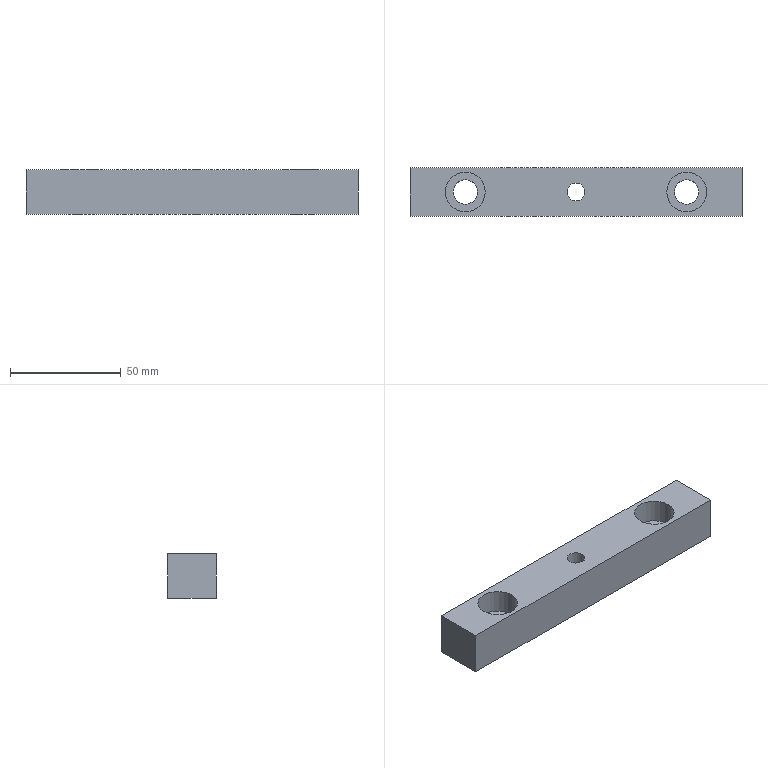Component | NX | DATUM_BLOCK | 1 solid | 13 faces | box 150 x 22 x 20 mm | volume 57750 mm3 | plane 8 | cylinder 5 | commonest cylinder face diameters 11 x2 18 x2 8 x1
STEP:
#1=CARTESIAN_POINT('',(0.,0.,0.));
#2=DIRECTION('',(0.,0.,1.));
#3=DIRECTION('',(1.,0.,0.));
#4=AXIS2_PLACEMENT_3D('',#1,#2,#3);
#5=CARTESIAN_POINT('',(-75.,-25.5,55.));
#6=VERTEX_POINT('',#5);
#7=CARTESIAN_POINT('',(-75.,-47.5,55.));
#8=VERTEX_POINT('',#7);
#9=CARTESIAN_POINT('',(-75.,-25.5,55.));
#10=DIRECTION('',(0.,-1.,0.));
#11=VECTOR('',#10,1.);
#12=LINE('',#9,#11);
#13=CARTESIAN_POINT('',(-75.,-25.5,35.));
#14=DIRECTION('',(-1.,0.,0.));
#15=DIRECTION('',(0.,0.,1.));
#16=AXIS2_PLACEMENT_3D('',#13,#14,#15);
#17=PLANE('',#16);
#18=CARTESIAN_POINT('',(20.,0.));
#19=DIRECTION('',(0.,-1.));
#20=VECTOR('',#19,1.);
#21=LINE('',#18,#20);
#22=(GEOMETRIC_REPRESENTATION_CONTEXT(2)PARAMETRIC_REPRESENTATION_CONTEXT()REPRESENTATION_CONTEXT('',''));
#23=DEFINITIONAL_REPRESENTATION('',(#21),#22);
#24=PCURVE('',#17,#23);
#25=CARTESIAN_POINT('',(0.,-36.5,55.));
#26=DIRECTION('',(0.,0.,1.));
#27=DIRECTION('',(1.,0.,0.));
#28=AXIS2_PLACEMENT_3D('',#25,#26,#27);
#29=PLANE('',#28);
#30=CARTESIAN_POINT('',(-75.,11.));
#31=DIRECTION('',(0.,-1.));
#32=VECTOR('',#31,1.);
#33=LINE('',#30,#32);
#34=(GEOMETRIC_REPRESENTATION_CONTEXT(2)PARAMETRIC_REPRESENTATION_CONTEXT()REPRESENTATION_CONTEXT('',''));
#35=DEFINITIONAL_REPRESENTATION('',(#33),#34);
#36=PCURVE('',#29,#35);
#37=SURFACE_CURVE('',#12,(#24,#36),.PCURVE_S1.);
#38=EDGE_CURVE('',#6,#8,#37,.T.);
#39=ORIENTED_EDGE('',*,*,#38,.F.);
#40=CARTESIAN_POINT('',(-75.,-25.5,35.));
#41=VERTEX_POINT('',#40);
#42=CARTESIAN_POINT('',(-75.,-25.5,35.));
#43=DIRECTION('',(0.,0.,1.));
#44=VECTOR('',#43,1.);
#45=LINE('',#42,#44);
#46=CARTESIAN_POINT('',(0.,0.));
#47=DIRECTION('',(1.,0.));
#48=VECTOR('',#47,1.);
#49=LINE('',#46,#48);
#50=(GEOMETRIC_REPRESENTATION_CONTEXT(2)PARAMETRIC_REPRESENTATION_CONTEXT()REPRESENTATION_CONTEXT('',''));
#51=DEFINITIONAL_REPRESENTATION('',(#49),#50);
#52=PCURVE('',#17,#51);
#53=CARTESIAN_POINT('',(75.,-25.5,35.));
#54=DIRECTION('',(0.,1.,0.));
#55=DIRECTION('',(0.,0.,1.));
#56=AXIS2_PLACEMENT_3D('',#53,#54,#55);
#57=PLANE('',#56);
#58=CARTESIAN_POINT('',(0.,-150.));
#59=DIRECTION('',(1.,0.));
#60=VECTOR('',#59,1.);
#61=LINE('',#58,#60);
#62=(GEOMETRIC_REPRESENTATION_CONTEXT(2)PARAMETRIC_REPRESENTATION_CONTEXT()REPRESENTATION_CONTEXT('',''));
#63=DEFINITIONAL_REPRESENTATION('',(#61),#62);
#64=PCURVE('',#57,#63);
#65=SURFACE_CURVE('',#45,(#52,#64),.PCURVE_S1.);
#66=EDGE_CURVE('',#41,#6,#65,.T.);
#67=ORIENTED_EDGE('',*,*,#66,.F.);
#68=CARTESIAN_POINT('',(-75.,-47.5,35.));
#69=VERTEX_POINT('',#68);
#70=CARTESIAN_POINT('',(-75.,-25.5,35.));
#71=DIRECTION('',(0.,-1.,0.));
#72=VECTOR('',#71,1.);
#73=LINE('',#70,#72);
#74=CARTESIAN_POINT('',(0.,0.));
#75=DIRECTION('',(0.,-1.));
#76=VECTOR('',#75,1.);
#77=LINE('',#74,#76);
#78=(GEOMETRIC_REPRESENTATION_CONTEXT(2)PARAMETRIC_REPRESENTATION_CONTEXT()REPRESENTATION_CONTEXT('',''));
#79=DEFINITIONAL_REPRESENTATION('',(#77),#78);
#80=PCURVE('',#17,#79);
#81=CARTESIAN_POINT('',(0.,-36.5,35.));
#82=DIRECTION('',(0.,0.,1.));
#83=DIRECTION('',(1.,0.,0.));
#84=AXIS2_PLACEMENT_3D('',#81,#82,#83);
#85=PLANE('',#84);
#86=CARTESIAN_POINT('',(-75.,11.));
#87=DIRECTION('',(0.,-1.));
#88=VECTOR('',#87,1.);
#89=LINE('',#86,#88);
#90=(GEOMETRIC_REPRESENTATION_CONTEXT(2)PARAMETRIC_REPRESENTATION_CONTEXT()REPRESENTATION_CONTEXT('',''));
#91=DEFINITIONAL_REPRESENTATION('',(#89),#90);
#92=PCURVE('',#85,#91);
#93=SURFACE_CURVE('',#73,(#80,#92),.PCURVE_S1.);
#94=EDGE_CURVE('',#41,#69,#93,.T.);
#95=ORIENTED_EDGE('',*,*,#94,.T.);
#96=CARTESIAN_POINT('',(-75.,-47.5,35.));
#97=DIRECTION('',(0.,0.,1.));
#98=VECTOR('',#97,1.);
#99=LINE('',#96,#98);
#100=CARTESIAN_POINT('',(0.,-22.));
#101=DIRECTION('',(1.,0.));
#102=VECTOR('',#101,1.);
#103=LINE('',#100,#102);
#104=(GEOMETRIC_REPRESENTATION_CONTEXT(2)PARAMETRIC_REPRESENTATION_CONTEXT()REPRESENTATION_CONTEXT('',''));
#105=DEFINITIONAL_REPRESENTATION('',(#103),#104);
#106=PCURVE('',#17,#105);
#107=CARTESIAN_POINT('',(-75.,-47.5,35.));
#108=DIRECTION('',(0.,-1.,0.));
#109=DIRECTION('',(0.,0.,-1.));
#110=AXIS2_PLACEMENT_3D('',#107,#108,#109);
#111=PLANE('',#110);
#112=CARTESIAN_POINT('',(0.,0.));
#113=DIRECTION('',(-1.,0.));
#114=VECTOR('',#113,1.);
#115=LINE('',#112,#114);
#116=(GEOMETRIC_REPRESENTATION_CONTEXT(2)PARAMETRIC_REPRESENTATION_CONTEXT()REPRESENTATION_CONTEXT('',''));
#117=DEFINITIONAL_REPRESENTATION('',(#115),#116);
#118=PCURVE('',#111,#117);
#119=SURFACE_CURVE('',#99,(#106,#118),.PCURVE_S1.);
#120=EDGE_CURVE('',#69,#8,#119,.T.);
#121=ORIENTED_EDGE('',*,*,#120,.T.);
#122=EDGE_LOOP('',(#39,#67,#95,#121));
#123=FACE_BOUND('',#122,.T.);
#124=ADVANCED_FACE('',(#123),#17,.T.);
#125=CARTESIAN_POINT('',(75.,-47.5,55.));
#126=VERTEX_POINT('',#125);
#127=CARTESIAN_POINT('',(-75.,-47.5,55.));
#128=DIRECTION('',(1.,0.,0.));
#129=VECTOR('',#128,1.);
#130=LINE('',#127,#129);
#131=CARTESIAN_POINT('',(-20.,0.));
#132=DIRECTION('',(0.,1.));
#133=VECTOR('',#132,1.);
#134=LINE('',#131,#133);
#135=(GEOMETRIC_REPRESENTATION_CONTEXT(2)PARAMETRIC_REPRESENTATION_CONTEXT()REPRESENTATION_CONTEXT('',''));
#136=DEFINITIONAL_REPRESENTATION('',(#134),#135);
#137=PCURVE('',#111,#136);
#138=CARTESIAN_POINT('',(-75.,-11.));
#139=DIRECTION('',(1.,0.));
#140=VECTOR('',#139,1.);
#141=LINE('',#138,#140);
#142=(GEOMETRIC_REPRESENTATION_CONTEXT(2)PARAMETRIC_REPRESENTATION_CONTEXT()REPRESENTATION_CONTEXT('',''));
#143=DEFINITIONAL_REPRESENTATION('',(#141),#142);
#144=PCURVE('',#29,#143);
#145=SURFACE_CURVE('',#130,(#137,#144),.PCURVE_S1.);
#146=EDGE_CURVE('',#8,#126,#145,.T.);
#147=ORIENTED_EDGE('',*,*,#146,.F.);
#148=ORIENTED_EDGE('',*,*,#120,.F.);
#149=CARTESIAN_POINT('',(75.,-47.5,35.));
#150=VERTEX_POINT('',#149);
#151=CARTESIAN_POINT('',(-75.,-47.5,35.));
#152=DIRECTION('',(1.,0.,0.));
#153=VECTOR('',#152,1.);
#154=LINE('',#151,#153);
#155=CARTESIAN_POINT('',(0.,0.));
#156=DIRECTION('',(0.,1.));
#157=VECTOR('',#156,1.);
#158=LINE('',#155,#157);
#159=(GEOMETRIC_REPRESENTATION_CONTEXT(2)PARAMETRIC_REPRESENTATION_CONTEXT()REPRESENTATION_CONTEXT('',''));
#160=DEFINITIONAL_REPRESENTATION('',(#158),#159);
#161=PCURVE('',#111,#160);
#162=CARTESIAN_POINT('',(-75.,-11.));
#163=DIRECTION('',(1.,0.));
#164=VECTOR('',#163,1.);
#165=LINE('',#162,#164);
#166=(GEOMETRIC_REPRESENTATION_CONTEXT(2)PARAMETRIC_REPRESENTATION_CONTEXT()REPRESENTATION_CONTEXT('',''));
#167=DEFINITIONAL_REPRESENTATION('',(#165),#166);
#168=PCURVE('',#85,#167);
#169=SURFACE_CURVE('',#154,(#161,#168),.PCURVE_S1.);
#170=EDGE_CURVE('',#69,#150,#169,.T.);
#171=ORIENTED_EDGE('',*,*,#170,.T.);
#172=CARTESIAN_POINT('',(75.,-47.5,35.));
#173=DIRECTION('',(0.,0.,1.));
#174=VECTOR('',#173,1.);
#175=LINE('',#172,#174);
#176=CARTESIAN_POINT('',(0.,150.));
#177=DIRECTION('',(-1.,0.));
#178=VECTOR('',#177,1.);
#179=LINE('',#176,#178);
#180=(GEOMETRIC_REPRESENTATION_CONTEXT(2)PARAMETRIC_REPRESENTATION_CONTEXT()REPRESENTATION_CONTEXT('',''));
#181=DEFINITIONAL_REPRESENTATION('',(#179),#180);
#182=PCURVE('',#111,#181);
#183=CARTESIAN_POINT('',(75.,-47.5,35.));
#184=DIRECTION('',(1.,0.,0.));
#185=DIRECTION('',(0.,0.,-1.));
#186=AXIS2_PLACEMENT_3D('',#183,#184,#185);
#187=PLANE('',#186);
#188=CARTESIAN_POINT('',(0.,0.));
#189=DIRECTION('',(-1.,0.));
#190=VECTOR('',#189,1.);
#191=LINE('',#188,#190);
#192=(GEOMETRIC_REPRESENTATION_CONTEXT(2)PARAMETRIC_REPRESENTATION_CONTEXT()REPRESENTATION_CONTEXT('',''));
#193=DEFINITIONAL_REPRESENTATION('',(#191),#192);
#194=PCURVE('',#187,#193);
#195=SURFACE_CURVE('',#175,(#182,#194),.PCURVE_S1.);
#196=EDGE_CURVE('',#150,#126,#195,.T.);
#197=ORIENTED_EDGE('',*,*,#196,.T.);
#198=EDGE_LOOP('',(#147,#148,#171,#197));
#199=FACE_BOUND('',#198,.T.);
#200=ADVANCED_FACE('',(#199),#111,.T.);
#201=CARTESIAN_POINT('',(75.,-25.5,55.));
#202=VERTEX_POINT('',#201);
#203=CARTESIAN_POINT('',(75.,-47.5,55.));
#204=DIRECTION('',(0.,1.,0.));
#205=VECTOR('',#204,1.);
#206=LINE('',#203,#205);
#207=CARTESIAN_POINT('',(-20.,0.));
#208=DIRECTION('',(0.,1.));
#209=VECTOR('',#208,1.);
#210=LINE('',#207,#209);
#211=(GEOMETRIC_REPRESENTATION_CONTEXT(2)PARAMETRIC_REPRESENTATION_CONTEXT()REPRESENTATION_CONTEXT('',''));
#212=DEFINITIONAL_REPRESENTATION('',(#210),#211);
#213=PCURVE('',#187,#212);
#214=CARTESIAN_POINT('',(75.,-11.));
#215=DIRECTION('',(0.,1.));
#216=VECTOR('',#215,1.);
#217=LINE('',#214,#216);
#218=(GEOMETRIC_REPRESENTATION_CONTEXT(2)PARAMETRIC_REPRESENTATION_CONTEXT()REPRESENTATION_CONTEXT('',''));
#219=DEFINITIONAL_REPRESENTATION('',(#217),#218);
#220=PCURVE('',#29,#219);
#221=SURFACE_CURVE('',#206,(#213,#220),.PCURVE_S1.);
#222=EDGE_CURVE('',#126,#202,#221,.T.);
#223=ORIENTED_EDGE('',*,*,#222,.F.);
#224=ORIENTED_EDGE('',*,*,#196,.F.);
#225=CARTESIAN_POINT('',(75.,-25.5,35.));
#226=VERTEX_POINT('',#225);
#227=CARTESIAN_POINT('',(75.,-47.5,35.));
#228=DIRECTION('',(0.,1.,0.));
#229=VECTOR('',#228,1.);
#230=LINE('',#227,#229);
#231=CARTESIAN_POINT('',(0.,0.));
#232=DIRECTION('',(0.,1.));
#233=VECTOR('',#232,1.);
#234=LINE('',#231,#233);
#235=(GEOMETRIC_REPRESENTATION_CONTEXT(2)PARAMETRIC_REPRESENTATION_CONTEXT()REPRESENTATION_CONTEXT('',''));
#236=DEFINITIONAL_REPRESENTATION('',(#234),#235);
#237=PCURVE('',#187,#236);
#238=CARTESIAN_POINT('',(75.,-11.));
#239=DIRECTION('',(0.,1.));
#240=VECTOR('',#239,1.);
#241=LINE('',#238,#240);
#242=(GEOMETRIC_REPRESENTATION_CONTEXT(2)PARAMETRIC_REPRESENTATION_CONTEXT()REPRESENTATION_CONTEXT('',''));
#243=DEFINITIONAL_REPRESENTATION('',(#241),#242);
#244=PCURVE('',#85,#243);
#245=SURFACE_CURVE('',#230,(#237,#244),.PCURVE_S1.);
#246=EDGE_CURVE('',#150,#226,#245,.T.);
#247=ORIENTED_EDGE('',*,*,#246,.T.);
#248=CARTESIAN_POINT('',(75.,-25.5,35.));
#249=DIRECTION('',(0.,0.,1.));
#250=VECTOR('',#249,1.);
#251=LINE('',#248,#250);
#252=CARTESIAN_POINT('',(0.,22.));
#253=DIRECTION('',(-1.,0.));
#254=VECTOR('',#253,1.);
#255=LINE('',#252,#254);
#256=(GEOMETRIC_REPRESENTATION_CONTEXT(2)PARAMETRIC_REPRESENTATION_CONTEXT()REPRESENTATION_CONTEXT('',''));
#257=DEFINITIONAL_REPRESENTATION('',(#255),#256);
#258=PCURVE('',#187,#257);
#259=CARTESIAN_POINT('',(0.,0.));
#260=DIRECTION('',(1.,0.));
#261=VECTOR('',#260,1.);
#262=LINE('',#259,#261);
#263=(GEOMETRIC_REPRESENTATION_CONTEXT(2)PARAMETRIC_REPRESENTATION_CONTEXT()REPRESENTATION_CONTEXT('',''));
#264=DEFINITIONAL_REPRESENTATION('',(#262),#263);
#265=PCURVE('',#57,#264);
#266=SURFACE_CURVE('',#251,(#258,#265),.PCURVE_S1.);
#267=EDGE_CURVE('',#226,#202,#266,.T.);
#268=ORIENTED_EDGE('',*,*,#267,.T.);
#269=EDGE_LOOP('',(#223,#224,#247,#268));
#270=FACE_BOUND('',#269,.T.);
#271=ADVANCED_FACE('',(#270),#187,.T.);
#272=CARTESIAN_POINT('',(75.,-25.5,55.));
#273=DIRECTION('',(-1.,0.,0.));
#274=VECTOR('',#273,1.);
#275=LINE('',#272,#274);
#276=CARTESIAN_POINT('',(20.,0.));
#277=DIRECTION('',(0.,-1.));
#278=VECTOR('',#277,1.);
#279=LINE('',#276,#278);
#280=(GEOMETRIC_REPRESENTATION_CONTEXT(2)PARAMETRIC_REPRESENTATION_CONTEXT()REPRESENTATION_CONTEXT('',''));
#281=DEFINITIONAL_REPRESENTATION('',(#279),#280);
#282=PCURVE('',#57,#281);
#283=CARTESIAN_POINT('',(75.,11.));
#284=DIRECTION('',(-1.,0.));
#285=VECTOR('',#284,1.);
#286=LINE('',#283,#285);
#287=(GEOMETRIC_REPRESENTATION_CONTEXT(2)PARAMETRIC_REPRESENTATION_CONTEXT()REPRESENTATION_CONTEXT('',''));
#288=DEFINITIONAL_REPRESENTATION('',(#286),#287);
#289=PCURVE('',#29,#288);
#290=SURFACE_CURVE('',#275,(#282,#289),.PCURVE_S1.);
#291=EDGE_CURVE('',#202,#6,#290,.T.);
#292=ORIENTED_EDGE('',*,*,#291,.F.);
#293=ORIENTED_EDGE('',*,*,#267,.F.);
#294=CARTESIAN_POINT('',(75.,-25.5,35.));
#295=DIRECTION('',(-1.,0.,0.));
#296=VECTOR('',#295,1.);
#297=LINE('',#294,#296);
#298=CARTESIAN_POINT('',(0.,0.));
#299=DIRECTION('',(0.,-1.));
#300=VECTOR('',#299,1.);
#301=LINE('',#298,#300);
#302=(GEOMETRIC_REPRESENTATION_CONTEXT(2)PARAMETRIC_REPRESENTATION_CONTEXT()REPRESENTATION_CONTEXT('',''));
#303=DEFINITIONAL_REPRESENTATION('',(#301),#302);
#304=PCURVE('',#57,#303);
#305=CARTESIAN_POINT('',(75.,11.));
#306=DIRECTION('',(-1.,0.));
#307=VECTOR('',#306,1.);
#308=LINE('',#305,#307);
#309=(GEOMETRIC_REPRESENTATION_CONTEXT(2)PARAMETRIC_REPRESENTATION_CONTEXT()REPRESENTATION_CONTEXT('',''));
#310=DEFINITIONAL_REPRESENTATION('',(#308),#309);
#311=PCURVE('',#85,#310);
#312=SURFACE_CURVE('',#297,(#304,#311),.PCURVE_S1.);
#313=EDGE_CURVE('',#226,#41,#312,.T.);
#314=ORIENTED_EDGE('',*,*,#313,.T.);
#315=ORIENTED_EDGE('',*,*,#66,.T.);
#316=EDGE_LOOP('',(#292,#293,#314,#315));
#317=FACE_BOUND('',#316,.T.);
#318=ADVANCED_FACE('',(#317),#57,.T.);
#319=CARTESIAN_POINT('',(4.,-36.5,35.));
#320=VERTEX_POINT('',#319);
#321=CARTESIAN_POINT('',(-4.,-36.5,35.));
#322=VERTEX_POINT('',#321);
#323=CARTESIAN_POINT('',(0.,-36.5,35.));
#324=DIRECTION('',(0.,0.,1.));
#325=DIRECTION('',(1.,0.,0.));
#326=AXIS2_PLACEMENT_3D('',#323,#324,#325);
#327=CIRCLE('',#326,4.);
#328=CARTESIAN_POINT('',(0.,0.));
#329=DIRECTION('',(1.,0.));
#330=AXIS2_PLACEMENT_2D('',#328,#329);
#331=CIRCLE('',#330,4.);
#332=(GEOMETRIC_REPRESENTATION_CONTEXT(2)PARAMETRIC_REPRESENTATION_CONTEXT()REPRESENTATION_CONTEXT('',''));
#333=DEFINITIONAL_REPRESENTATION('',(#331),#332);
#334=PCURVE('',#85,#333);
#335=CARTESIAN_POINT('',(0.,-36.5,55.));
#336=DIRECTION('',(0.,0.,-1.));
#337=DIRECTION('',(-1.,0.,0.));
#338=AXIS2_PLACEMENT_3D('',#335,#336,#337);
#339=CYLINDRICAL_SURFACE('',#338,4.);
#340=CARTESIAN_POINT('',(3.142,20.));
#341=DIRECTION('',(-1.,0.));
#342=VECTOR('',#341,1.);
#343=LINE('',#340,#342);
#344=(GEOMETRIC_REPRESENTATION_CONTEXT(2)PARAMETRIC_REPRESENTATION_CONTEXT()REPRESENTATION_CONTEXT('',''));
#345=DEFINITIONAL_REPRESENTATION('',(#343),#344);
#346=PCURVE('',#339,#345);
#347=SURFACE_CURVE('',#327,(#334,#346),.PCURVE_S1.);
#348=EDGE_CURVE('',#320,#322,#347,.T.);
#349=ORIENTED_EDGE('',*,*,#348,.T.);
#350=CARTESIAN_POINT('',(0.,-36.5,35.));
#351=DIRECTION('',(0.,0.,1.));
#352=DIRECTION('',(1.,0.,0.));
#353=AXIS2_PLACEMENT_3D('',#350,#351,#352);
#354=CIRCLE('',#353,4.);
#355=CARTESIAN_POINT('',(0.,0.));
#356=DIRECTION('',(1.,0.));
#357=AXIS2_PLACEMENT_2D('',#355,#356);
#358=CIRCLE('',#357,4.);
#359=(GEOMETRIC_REPRESENTATION_CONTEXT(2)PARAMETRIC_REPRESENTATION_CONTEXT()REPRESENTATION_CONTEXT('',''));
#360=DEFINITIONAL_REPRESENTATION('',(#358),#359);
#361=PCURVE('',#85,#360);
#362=CARTESIAN_POINT('',(9.425,20.));
#363=DIRECTION('',(-1.,0.));
#364=VECTOR('',#363,1.);
#365=LINE('',#362,#364);
#366=(GEOMETRIC_REPRESENTATION_CONTEXT(2)PARAMETRIC_REPRESENTATION_CONTEXT()REPRESENTATION_CONTEXT('',''));
#367=DEFINITIONAL_REPRESENTATION('',(#365),#366);
#368=PCURVE('',#339,#367);
#369=SURFACE_CURVE('',#354,(#361,#368),.PCURVE_S1.);
#370=EDGE_CURVE('',#322,#320,#369,.T.);
#371=ORIENTED_EDGE('',*,*,#370,.T.);
#372=EDGE_LOOP('',(#349,#371));
#373=FACE_BOUND('',#372,.T.);
#374=CARTESIAN_POINT('',(55.5,-36.5,35.));
#375=VERTEX_POINT('',#374);
#376=CARTESIAN_POINT('',(44.5,-36.5,35.));
#377=VERTEX_POINT('',#376);
#378=CARTESIAN_POINT('',(50.,-36.5,35.));
#379=DIRECTION('',(0.,0.,1.));
#380=DIRECTION('',(1.,0.,0.));
#381=AXIS2_PLACEMENT_3D('',#378,#379,#380);
#382=CIRCLE('',#381,5.5);
#383=CARTESIAN_POINT('',(50.,0.));
#384=DIRECTION('',(1.,0.));
#385=AXIS2_PLACEMENT_2D('',#383,#384);
#386=CIRCLE('',#385,5.5);
#387=(GEOMETRIC_REPRESENTATION_CONTEXT(2)PARAMETRIC_REPRESENTATION_CONTEXT()REPRESENTATION_CONTEXT('',''));
#388=DEFINITIONAL_REPRESENTATION('',(#386),#387);
#389=PCURVE('',#85,#388);
#390=CARTESIAN_POINT('',(50.,-36.5,-22.629));
#391=DIRECTION('',(0.,0.,-1.));
#392=DIRECTION('',(-1.,0.,0.));
#393=AXIS2_PLACEMENT_3D('',#390,#391,#392);
#394=CYLINDRICAL_SURFACE('',#393,5.5);
#395=CARTESIAN_POINT('',(3.142,-57.629));
#396=DIRECTION('',(-1.,0.));
#397=VECTOR('',#396,1.);
#398=LINE('',#395,#397);
#399=(GEOMETRIC_REPRESENTATION_CONTEXT(2)PARAMETRIC_REPRESENTATION_CONTEXT()REPRESENTATION_CONTEXT('',''));
#400=DEFINITIONAL_REPRESENTATION('',(#398),#399);
#401=PCURVE('',#394,#400);
#402=SURFACE_CURVE('',#382,(#389,#401),.PCURVE_S1.);
#403=EDGE_CURVE('',#375,#377,#402,.T.);
#404=ORIENTED_EDGE('',*,*,#403,.T.);
#405=CARTESIAN_POINT('',(50.,-36.5,35.));
#406=DIRECTION('',(0.,0.,1.));
#407=DIRECTION('',(1.,0.,0.));
#408=AXIS2_PLACEMENT_3D('',#405,#406,#407);
#409=CIRCLE('',#408,5.5);
#410=CARTESIAN_POINT('',(50.,0.));
#411=DIRECTION('',(1.,0.));
#412=AXIS2_PLACEMENT_2D('',#410,#411);
#413=CIRCLE('',#412,5.5);
#414=(GEOMETRIC_REPRESENTATION_CONTEXT(2)PARAMETRIC_REPRESENTATION_CONTEXT()REPRESENTATION_CONTEXT('',''));
#415=DEFINITIONAL_REPRESENTATION('',(#413),#414);
#416=PCURVE('',#85,#415);
#417=CARTESIAN_POINT('',(9.425,-57.629));
#418=DIRECTION('',(-1.,0.));
#419=VECTOR('',#418,1.);
#420=LINE('',#417,#419);
#421=(GEOMETRIC_REPRESENTATION_CONTEXT(2)PARAMETRIC_REPRESENTATION_CONTEXT()REPRESENTATION_CONTEXT('',''));
#422=DEFINITIONAL_REPRESENTATION('',(#420),#421);
#423=PCURVE('',#394,#422);
#424=SURFACE_CURVE('',#409,(#416,#423),.PCURVE_S1.);
#425=EDGE_CURVE('',#377,#375,#424,.T.);
#426=ORIENTED_EDGE('',*,*,#425,.T.);
#427=EDGE_LOOP('',(#404,#426));
#428=FACE_BOUND('',#427,.T.);
#429=CARTESIAN_POINT('',(-44.5,-36.5,35.));
#430=VERTEX_POINT('',#429);
#431=CARTESIAN_POINT('',(-55.5,-36.5,35.));
#432=VERTEX_POINT('',#431);
#433=CARTESIAN_POINT('',(-50.,-36.5,35.));
#434=DIRECTION('',(0.,0.,1.));
#435=DIRECTION('',(1.,0.,0.));
#436=AXIS2_PLACEMENT_3D('',#433,#434,#435);
#437=CIRCLE('',#436,5.5);
#438=CARTESIAN_POINT('',(-50.,0.));
#439=DIRECTION('',(1.,0.));
#440=AXIS2_PLACEMENT_2D('',#438,#439);
#441=CIRCLE('',#440,5.5);
#442=(GEOMETRIC_REPRESENTATION_CONTEXT(2)PARAMETRIC_REPRESENTATION_CONTEXT()REPRESENTATION_CONTEXT('',''));
#443=DEFINITIONAL_REPRESENTATION('',(#441),#442);
#444=PCURVE('',#85,#443);
#445=CARTESIAN_POINT('',(-50.,-36.5,-22.629));
#446=DIRECTION('',(0.,0.,-1.));
#447=DIRECTION('',(-1.,0.,0.));
#448=AXIS2_PLACEMENT_3D('',#445,#446,#447);
#449=CYLINDRICAL_SURFACE('',#448,5.5);
#450=CARTESIAN_POINT('',(3.142,-57.629));
#451=DIRECTION('',(-1.,0.));
#452=VECTOR('',#451,1.);
#453=LINE('',#450,#452);
#454=(GEOMETRIC_REPRESENTATION_CONTEXT(2)PARAMETRIC_REPRESENTATION_CONTEXT()REPRESENTATION_CONTEXT('',''));
#455=DEFINITIONAL_REPRESENTATION('',(#453),#454);
#456=PCURVE('',#449,#455);
#457=SURFACE_CURVE('',#437,(#444,#456),.PCURVE_S1.);
#458=EDGE_CURVE('',#430,#432,#457,.T.);
#459=ORIENTED_EDGE('',*,*,#458,.T.);
#460=CARTESIAN_POINT('',(-50.,-36.5,35.));
#461=DIRECTION('',(0.,0.,1.));
#462=DIRECTION('',(1.,0.,0.));
#463=AXIS2_PLACEMENT_3D('',#460,#461,#462);
#464=CIRCLE('',#463,5.5);
#465=CARTESIAN_POINT('',(-50.,0.));
#466=DIRECTION('',(1.,0.));
#467=AXIS2_PLACEMENT_2D('',#465,#466);
#468=CIRCLE('',#467,5.5);
#469=(GEOMETRIC_REPRESENTATION_CONTEXT(2)PARAMETRIC_REPRESENTATION_CONTEXT()REPRESENTATION_CONTEXT('',''));
#470=DEFINITIONAL_REPRESENTATION('',(#468),#469);
#471=PCURVE('',#85,#470);
#472=CARTESIAN_POINT('',(9.425,-57.629));
#473=DIRECTION('',(-1.,0.));
#474=VECTOR('',#473,1.);
#475=LINE('',#472,#474);
#476=(GEOMETRIC_REPRESENTATION_CONTEXT(2)PARAMETRIC_REPRESENTATION_CONTEXT()REPRESENTATION_CONTEXT('',''));
#477=DEFINITIONAL_REPRESENTATION('',(#475),#476);
#478=PCURVE('',#449,#477);
#479=SURFACE_CURVE('',#464,(#471,#478),.PCURVE_S1.);
#480=EDGE_CURVE('',#432,#430,#479,.T.);
#481=ORIENTED_EDGE('',*,*,#480,.T.);
#482=EDGE_LOOP('',(#459,#481));
#483=FACE_BOUND('',#482,.T.);
#484=ORIENTED_EDGE('',*,*,#94,.F.);
#485=ORIENTED_EDGE('',*,*,#313,.F.);
#486=ORIENTED_EDGE('',*,*,#246,.F.);
#487=ORIENTED_EDGE('',*,*,#170,.F.);
#488=EDGE_LOOP('',(#484,#485,#486,#487));
#489=FACE_BOUND('',#488,.T.);
#490=ADVANCED_FACE('',(#373,#428,#483,#489),#85,.F.);
#491=CARTESIAN_POINT('',(-4.,-36.5,55.));
#492=VERTEX_POINT('',#491);
#493=CARTESIAN_POINT('',(0.,-36.5,55.));
#494=DIRECTION('',(0.,0.,-1.));
#495=DIRECTION('',(-1.,0.,0.));
#496=AXIS2_PLACEMENT_3D('',#493,#494,#495);
#497=CIRCLE('',#496,4.);
#498=CARTESIAN_POINT('',(-4.,0.));
#499=CARTESIAN_POINT('',(-4.,6.928));
#500=CARTESIAN_POINT('',(2.,3.464));
#501=CARTESIAN_POINT('',(8.,0.));
#502=CARTESIAN_POINT('',(2.,-3.464));
#503=CARTESIAN_POINT('',(-4.,-6.928));
#504=CARTESIAN_POINT('',(-4.,0.));
#505=(BOUNDED_CURVE()B_SPLINE_CURVE(2,(#498,#499,#500,#501,#502,#503,#504),.UNSPECIFIED.,.T.,.F.)B_SPLINE_CURVE_WITH_KNOTS((1,2,2,2,2,1),(-2.094,0.,2.094,4.189,6.283,8.378),.UNSPECIFIED.)CURVE()GEOMETRIC_REPRESENTATION_ITEM()RATIONAL_B_SPLINE_CURVE((1.,0.5,1.,0.5,1.,0.5,1.))REPRESENTATION_ITEM(''));
#506=(GEOMETRIC_REPRESENTATION_CONTEXT(2)PARAMETRIC_REPRESENTATION_CONTEXT()REPRESENTATION_CONTEXT('',''));
#507=DEFINITIONAL_REPRESENTATION('',(#505),#506);
#508=PCURVE('',#29,#507);
#509=CARTESIAN_POINT('',(0.,0.));
#510=DIRECTION('',(1.,0.));
#511=VECTOR('',#510,1.);
#512=LINE('',#509,#511);
#513=(GEOMETRIC_REPRESENTATION_CONTEXT(2)PARAMETRIC_REPRESENTATION_CONTEXT()REPRESENTATION_CONTEXT('',''));
#514=DEFINITIONAL_REPRESENTATION('',(#512),#513);
#515=PCURVE('',#339,#514);
#516=SURFACE_CURVE('',#497,(#508,#515),.PCURVE_S1.);
#517=EDGE_CURVE('',#492,#492,#516,.T.);
#518=ORIENTED_EDGE('',*,*,#517,.T.);
#519=EDGE_LOOP('',(#518));
#520=FACE_BOUND('',#519,.T.);
#521=CARTESIAN_POINT('',(41.,-36.5,55.));
#522=VERTEX_POINT('',#521);
#523=CARTESIAN_POINT('',(50.,-36.5,55.));
#524=DIRECTION('',(0.,0.,-1.));
#525=DIRECTION('',(-1.,0.,0.));
#526=AXIS2_PLACEMENT_3D('',#523,#524,#525);
#527=CIRCLE('',#526,9.);
#528=CARTESIAN_POINT('',(41.,0.));
#529=CARTESIAN_POINT('',(41.,15.588));
#530=CARTESIAN_POINT('',(54.5,7.794));
#531=CARTESIAN_POINT('',(68.,0.));
#532=CARTESIAN_POINT('',(54.5,-7.794));
#533=CARTESIAN_POINT('',(41.,-15.588));
#534=CARTESIAN_POINT('',(41.,0.));
#535=(BOUNDED_CURVE()B_SPLINE_CURVE(2,(#528,#529,#530,#531,#532,#533,#534),.UNSPECIFIED.,.T.,.F.)B_SPLINE_CURVE_WITH_KNOTS((1,2,2,2,2,1),(-2.094,0.,2.094,4.189,6.283,8.378),.UNSPECIFIED.)CURVE()GEOMETRIC_REPRESENTATION_ITEM()RATIONAL_B_SPLINE_CURVE((1.,0.5,1.,0.5,1.,0.5,1.))REPRESENTATION_ITEM(''));
#536=(GEOMETRIC_REPRESENTATION_CONTEXT(2)PARAMETRIC_REPRESENTATION_CONTEXT()REPRESENTATION_CONTEXT('',''));
#537=DEFINITIONAL_REPRESENTATION('',(#535),#536);
#538=PCURVE('',#29,#537);
#539=CARTESIAN_POINT('',(50.,-36.5,55.));
#540=DIRECTION('',(0.,0.,-1.));
#541=DIRECTION('',(-1.,0.,0.));
#542=AXIS2_PLACEMENT_3D('',#539,#540,#541);
#543=CYLINDRICAL_SURFACE('',#542,9.);
#544=CARTESIAN_POINT('',(0.,0.));
#545=DIRECTION('',(1.,0.));
#546=VECTOR('',#545,1.);
#547=LINE('',#544,#546);
#548=(GEOMETRIC_REPRESENTATION_CONTEXT(2)PARAMETRIC_REPRESENTATION_CONTEXT()REPRESENTATION_CONTEXT('',''));
#549=DEFINITIONAL_REPRESENTATION('',(#547),#548);
#550=PCURVE('',#543,#549);
#551=SURFACE_CURVE('',#527,(#538,#550),.PCURVE_S1.);
#552=EDGE_CURVE('',#522,#522,#551,.T.);
#553=ORIENTED_EDGE('',*,*,#552,.T.);
#554=EDGE_LOOP('',(#553));
#555=FACE_BOUND('',#554,.T.);
#556=CARTESIAN_POINT('',(-59.,-36.5,55.));
#557=VERTEX_POINT('',#556);
#558=CARTESIAN_POINT('',(-50.,-36.5,55.));
#559=DIRECTION('',(0.,0.,-1.));
#560=DIRECTION('',(-1.,0.,0.));
#561=AXIS2_PLACEMENT_3D('',#558,#559,#560);
#562=CIRCLE('',#561,9.);
#563=CARTESIAN_POINT('',(-59.,0.));
#564=CARTESIAN_POINT('',(-59.,15.588));
#565=CARTESIAN_POINT('',(-45.5,7.794));
#566=CARTESIAN_POINT('',(-32.,0.));
#567=CARTESIAN_POINT('',(-45.5,-7.794));
#568=CARTESIAN_POINT('',(-59.,-15.588));
#569=CARTESIAN_POINT('',(-59.,0.));
#570=(BOUNDED_CURVE()B_SPLINE_CURVE(2,(#563,#564,#565,#566,#567,#568,#569),.UNSPECIFIED.,.T.,.F.)B_SPLINE_CURVE_WITH_KNOTS((1,2,2,2,2,1),(-2.094,0.,2.094,4.189,6.283,8.378),.UNSPECIFIED.)CURVE()GEOMETRIC_REPRESENTATION_ITEM()RATIONAL_B_SPLINE_CURVE((1.,0.5,1.,0.5,1.,0.5,1.))REPRESENTATION_ITEM(''));
#571=(GEOMETRIC_REPRESENTATION_CONTEXT(2)PARAMETRIC_REPRESENTATION_CONTEXT()REPRESENTATION_CONTEXT('',''));
#572=DEFINITIONAL_REPRESENTATION('',(#570),#571);
#573=PCURVE('',#29,#572);
#574=CARTESIAN_POINT('',(-50.,-36.5,55.));
#575=DIRECTION('',(0.,0.,-1.));
#576=DIRECTION('',(-1.,0.,0.));
#577=AXIS2_PLACEMENT_3D('',#574,#575,#576);
#578=CYLINDRICAL_SURFACE('',#577,9.);
#579=CARTESIAN_POINT('',(0.,0.));
#580=DIRECTION('',(1.,0.));
#581=VECTOR('',#580,1.);
#582=LINE('',#579,#581);
#583=(GEOMETRIC_REPRESENTATION_CONTEXT(2)PARAMETRIC_REPRESENTATION_CONTEXT()REPRESENTATION_CONTEXT('',''));
#584=DEFINITIONAL_REPRESENTATION('',(#582),#583);
#585=PCURVE('',#578,#584);
#586=SURFACE_CURVE('',#562,(#573,#585),.PCURVE_S1.);
#587=EDGE_CURVE('',#557,#557,#586,.T.);
#588=ORIENTED_EDGE('',*,*,#587,.T.);
#589=EDGE_LOOP('',(#588));
#590=FACE_BOUND('',#589,.T.);
#591=ORIENTED_EDGE('',*,*,#38,.T.);
#592=ORIENTED_EDGE('',*,*,#146,.T.);
#593=ORIENTED_EDGE('',*,*,#222,.T.);
#594=ORIENTED_EDGE('',*,*,#291,.T.);
#595=EDGE_LOOP('',(#591,#592,#593,#594));
#596=FACE_BOUND('',#595,.T.);
#597=ADVANCED_FACE('',(#520,#555,#590,#596),#29,.T.);
#598=CARTESIAN_POINT('',(-55.5,-36.5,44.2));
#599=VERTEX_POINT('',#598);
#600=CARTESIAN_POINT('',(-50.,-36.5,44.2));
#601=DIRECTION('',(0.,0.,1.));
#602=DIRECTION('',(-1.,0.,0.));
#603=AXIS2_PLACEMENT_3D('',#600,#601,#602);
#604=CIRCLE('',#603,5.5);
#605=CARTESIAN_POINT('',(6.283,-66.829));
#606=DIRECTION('',(-1.,0.));
#607=VECTOR('',#606,1.);
#608=LINE('',#605,#607);
#609=(GEOMETRIC_REPRESENTATION_CONTEXT(2)PARAMETRIC_REPRESENTATION_CONTEXT()REPRESENTATION_CONTEXT('',''));
#610=DEFINITIONAL_REPRESENTATION('',(#608),#609);
#611=PCURVE('',#449,#610);
#612=CARTESIAN_POINT('',(-50.,-36.5,44.2));
#613=DIRECTION('',(0.,0.,-1.));
#614=DIRECTION('',(-1.,0.,0.));
#615=AXIS2_PLACEMENT_3D('',#612,#613,#614);
#616=PLANE('',#615);
#617=CARTESIAN_POINT('',(5.5,0.));
#618=CARTESIAN_POINT('',(5.5,-9.526));
#619=CARTESIAN_POINT('',(-2.75,-4.763));
#620=CARTESIAN_POINT('',(-11.,-0.));
#621=CARTESIAN_POINT('',(-2.75,4.763));
#622=CARTESIAN_POINT('',(5.5,9.526));
#623=CARTESIAN_POINT('',(5.5,0.));
#624=(BOUNDED_CURVE()B_SPLINE_CURVE(2,(#617,#618,#619,#620,#621,#622,#623),.UNSPECIFIED.,.T.,.F.)B_SPLINE_CURVE_WITH_KNOTS((1,2,2,2,2,1),(-2.094,0.,2.094,4.189,6.283,8.378),.UNSPECIFIED.)CURVE()GEOMETRIC_REPRESENTATION_ITEM()RATIONAL_B_SPLINE_CURVE((1.,0.5,1.,0.5,1.,0.5,1.))REPRESENTATION_ITEM(''));
#625=(GEOMETRIC_REPRESENTATION_CONTEXT(2)PARAMETRIC_REPRESENTATION_CONTEXT()REPRESENTATION_CONTEXT('',''));
#626=DEFINITIONAL_REPRESENTATION('',(#624),#625);
#627=PCURVE('',#616,#626);
#628=SURFACE_CURVE('',#604,(#611,#627),.PCURVE_S1.);
#629=EDGE_CURVE('',#599,#599,#628,.T.);
#630=ORIENTED_EDGE('',*,*,#629,.F.);
#631=CARTESIAN_POINT('',(-55.5,-36.5,44.2));
#632=CARTESIAN_POINT('',(-55.5,-36.5,35.));
#633=B_SPLINE_CURVE_WITH_KNOTS('',1,(#631,#632),.UNSPECIFIED.,.F.,.F.,(2,2),(-66.829,-57.629),.PIECEWISE_BEZIER_KNOTS.);
#634=CARTESIAN_POINT('',(6.283,0.));
#635=DIRECTION('',(0.,1.));
#636=VECTOR('',#635,1.);
#637=LINE('',#634,#636);
#638=(GEOMETRIC_REPRESENTATION_CONTEXT(2)PARAMETRIC_REPRESENTATION_CONTEXT()REPRESENTATION_CONTEXT('',''));
#639=DEFINITIONAL_REPRESENTATION('',(#637),#638);
#640=PCURVE('',#449,#639);
#641=CARTESIAN_POINT('',(0.,0.));
#642=DIRECTION('',(0.,1.));
#643=VECTOR('',#642,1.);
#644=LINE('',#641,#643);
#645=(GEOMETRIC_REPRESENTATION_CONTEXT(2)PARAMETRIC_REPRESENTATION_CONTEXT()REPRESENTATION_CONTEXT('',''));
#646=DEFINITIONAL_REPRESENTATION('',(#644),#645);
#647=PCURVE('',#449,#646);
#648=SEAM_CURVE('',#633,(#640,#647),.PCURVE_S1.);
#649=EDGE_CURVE('',#599,#432,#648,.T.);
#650=ORIENTED_EDGE('',*,*,#649,.T.);
#651=ORIENTED_EDGE('',*,*,#480,.T.);
#652=ORIENTED_EDGE('',*,*,#458,.T.);
#653=ORIENTED_EDGE('',*,*,#649,.F.);
#654=EDGE_LOOP('',(#630,#650,#651,#652,#653));
#655=FACE_BOUND('',#654,.F.);
#656=ADVANCED_FACE('',(#655),#449,.F.);
#657=ORIENTED_EDGE('',*,*,#629,.F.);
#658=EDGE_LOOP('',(#657));
#659=FACE_BOUND('',#658,.T.);
#660=CARTESIAN_POINT('',(-59.,-36.5,44.2));
#661=VERTEX_POINT('',#660);
#662=CARTESIAN_POINT('',(-50.,-36.5,44.2));
#663=DIRECTION('',(0.,0.,1.));
#664=DIRECTION('',(-1.,0.,0.));
#665=AXIS2_PLACEMENT_3D('',#662,#663,#664);
#666=CIRCLE('',#665,9.);
#667=CARTESIAN_POINT('',(9.,0.));
#668=CARTESIAN_POINT('',(9.,-15.588));
#669=CARTESIAN_POINT('',(-4.5,-7.794));
#670=CARTESIAN_POINT('',(-18.,-0.));
#671=CARTESIAN_POINT('',(-4.5,7.794));
#672=CARTESIAN_POINT('',(9.,15.588));
#673=CARTESIAN_POINT('',(9.,0.));
#674=(BOUNDED_CURVE()B_SPLINE_CURVE(2,(#667,#668,#669,#670,#671,#672,#673),.UNSPECIFIED.,.T.,.F.)B_SPLINE_CURVE_WITH_KNOTS((1,2,2,2,2,1),(-2.094,0.,2.094,4.189,6.283,8.378),.UNSPECIFIED.)CURVE()GEOMETRIC_REPRESENTATION_ITEM()RATIONAL_B_SPLINE_CURVE((1.,0.5,1.,0.5,1.,0.5,1.))REPRESENTATION_ITEM(''));
#675=(GEOMETRIC_REPRESENTATION_CONTEXT(2)PARAMETRIC_REPRESENTATION_CONTEXT()REPRESENTATION_CONTEXT('',''));
#676=DEFINITIONAL_REPRESENTATION('',(#674),#675);
#677=PCURVE('',#616,#676);
#678=CARTESIAN_POINT('',(6.283,10.8));
#679=DIRECTION('',(-1.,0.));
#680=VECTOR('',#679,1.);
#681=LINE('',#678,#680);
#682=(GEOMETRIC_REPRESENTATION_CONTEXT(2)PARAMETRIC_REPRESENTATION_CONTEXT()REPRESENTATION_CONTEXT('',''));
#683=DEFINITIONAL_REPRESENTATION('',(#681),#682);
#684=PCURVE('',#578,#683);
#685=SURFACE_CURVE('',#666,(#677,#684),.PCURVE_S1.);
#686=EDGE_CURVE('',#661,#661,#685,.T.);
#687=ORIENTED_EDGE('',*,*,#686,.T.);
#688=EDGE_LOOP('',(#687));
#689=FACE_BOUND('',#688,.T.);
#690=ADVANCED_FACE('',(#659,#689),#616,.F.);
#691=ORIENTED_EDGE('',*,*,#686,.T.);
#692=CARTESIAN_POINT('',(-59.,-36.5,55.));
#693=CARTESIAN_POINT('',(-59.,-36.5,44.2));
#694=B_SPLINE_CURVE_WITH_KNOTS('',1,(#692,#693),.UNSPECIFIED.,.F.,.F.,(2,2),(0.,10.8),.PIECEWISE_BEZIER_KNOTS.);
#695=CARTESIAN_POINT('',(0.,0.));
#696=DIRECTION('',(0.,1.));
#697=VECTOR('',#696,1.);
#698=LINE('',#695,#697);
#699=(GEOMETRIC_REPRESENTATION_CONTEXT(2)PARAMETRIC_REPRESENTATION_CONTEXT()REPRESENTATION_CONTEXT('',''));
#700=DEFINITIONAL_REPRESENTATION('',(#698),#699);
#701=PCURVE('',#578,#700);
#702=CARTESIAN_POINT('',(6.283,0.));
#703=DIRECTION('',(0.,1.));
#704=VECTOR('',#703,1.);
#705=LINE('',#702,#704);
#706=(GEOMETRIC_REPRESENTATION_CONTEXT(2)PARAMETRIC_REPRESENTATION_CONTEXT()REPRESENTATION_CONTEXT('',''));
#707=DEFINITIONAL_REPRESENTATION('',(#705),#706);
#708=PCURVE('',#578,#707);
#709=SEAM_CURVE('',#694,(#701,#708),.PCURVE_S1.);
#710=EDGE_CURVE('',#557,#661,#709,.T.);
#711=ORIENTED_EDGE('',*,*,#710,.F.);
#712=ORIENTED_EDGE('',*,*,#587,.T.);
#713=ORIENTED_EDGE('',*,*,#710,.T.);
#714=EDGE_LOOP('',(#691,#711,#712,#713));
#715=FACE_BOUND('',#714,.F.);
#716=ADVANCED_FACE('',(#715),#578,.F.);
#717=CARTESIAN_POINT('',(44.5,-36.5,44.2));
#718=VERTEX_POINT('',#717);
#719=CARTESIAN_POINT('',(50.,-36.5,44.2));
#720=DIRECTION('',(0.,0.,1.));
#721=DIRECTION('',(-1.,0.,0.));
#722=AXIS2_PLACEMENT_3D('',#719,#720,#721);
#723=CIRCLE('',#722,5.5);
#724=CARTESIAN_POINT('',(6.283,-66.829));
#725=DIRECTION('',(-1.,0.));
#726=VECTOR('',#725,1.);
#727=LINE('',#724,#726);
#728=(GEOMETRIC_REPRESENTATION_CONTEXT(2)PARAMETRIC_REPRESENTATION_CONTEXT()REPRESENTATION_CONTEXT('',''));
#729=DEFINITIONAL_REPRESENTATION('',(#727),#728);
#730=PCURVE('',#394,#729);
#731=CARTESIAN_POINT('',(50.,-36.5,44.2));
#732=DIRECTION('',(0.,0.,-1.));
#733=DIRECTION('',(-1.,0.,0.));
#734=AXIS2_PLACEMENT_3D('',#731,#732,#733);
#735=PLANE('',#734);
#736=CARTESIAN_POINT('',(5.5,0.));
#737=CARTESIAN_POINT('',(5.5,-9.526));
#738=CARTESIAN_POINT('',(-2.75,-4.763));
#739=CARTESIAN_POINT('',(-11.,-0.));
#740=CARTESIAN_POINT('',(-2.75,4.763));
#741=CARTESIAN_POINT('',(5.5,9.526));
#742=CARTESIAN_POINT('',(5.5,0.));
#743=(BOUNDED_CURVE()B_SPLINE_CURVE(2,(#736,#737,#738,#739,#740,#741,#742),.UNSPECIFIED.,.T.,.F.)B_SPLINE_CURVE_WITH_KNOTS((1,2,2,2,2,1),(-2.094,0.,2.094,4.189,6.283,8.378),.UNSPECIFIED.)CURVE()GEOMETRIC_REPRESENTATION_ITEM()RATIONAL_B_SPLINE_CURVE((1.,0.5,1.,0.5,1.,0.5,1.))REPRESENTATION_ITEM(''));
#744=(GEOMETRIC_REPRESENTATION_CONTEXT(2)PARAMETRIC_REPRESENTATION_CONTEXT()REPRESENTATION_CONTEXT('',''));
#745=DEFINITIONAL_REPRESENTATION('',(#743),#744);
#746=PCURVE('',#735,#745);
#747=SURFACE_CURVE('',#723,(#730,#746),.PCURVE_S1.);
#748=EDGE_CURVE('',#718,#718,#747,.T.);
#749=ORIENTED_EDGE('',*,*,#748,.F.);
#750=CARTESIAN_POINT('',(44.5,-36.5,44.2));
#751=CARTESIAN_POINT('',(44.5,-36.5,35.));
#752=B_SPLINE_CURVE_WITH_KNOTS('',1,(#750,#751),.UNSPECIFIED.,.F.,.F.,(2,2),(-66.829,-57.629),.PIECEWISE_BEZIER_KNOTS.);
#753=CARTESIAN_POINT('',(6.283,0.));
#754=DIRECTION('',(0.,1.));
#755=VECTOR('',#754,1.);
#756=LINE('',#753,#755);
#757=(GEOMETRIC_REPRESENTATION_CONTEXT(2)PARAMETRIC_REPRESENTATION_CONTEXT()REPRESENTATION_CONTEXT('',''));
#758=DEFINITIONAL_REPRESENTATION('',(#756),#757);
#759=PCURVE('',#394,#758);
#760=CARTESIAN_POINT('',(0.,0.));
#761=DIRECTION('',(0.,1.));
#762=VECTOR('',#761,1.);
#763=LINE('',#760,#762);
#764=(GEOMETRIC_REPRESENTATION_CONTEXT(2)PARAMETRIC_REPRESENTATION_CONTEXT()REPRESENTATION_CONTEXT('',''));
#765=DEFINITIONAL_REPRESENTATION('',(#763),#764);
#766=PCURVE('',#394,#765);
#767=SEAM_CURVE('',#752,(#759,#766),.PCURVE_S1.);
#768=EDGE_CURVE('',#718,#377,#767,.T.);
#769=ORIENTED_EDGE('',*,*,#768,.T.);
#770=ORIENTED_EDGE('',*,*,#425,.T.);
#771=ORIENTED_EDGE('',*,*,#403,.T.);
#772=ORIENTED_EDGE('',*,*,#768,.F.);
#773=EDGE_LOOP('',(#749,#769,#770,#771,#772));
#774=FACE_BOUND('',#773,.F.);
#775=ADVANCED_FACE('',(#774),#394,.F.);
#776=ORIENTED_EDGE('',*,*,#748,.F.);
#777=EDGE_LOOP('',(#776));
#778=FACE_BOUND('',#777,.T.);
#779=CARTESIAN_POINT('',(41.,-36.5,44.2));
#780=VERTEX_POINT('',#779);
#781=CARTESIAN_POINT('',(50.,-36.5,44.2));
#782=DIRECTION('',(0.,0.,1.));
#783=DIRECTION('',(-1.,0.,0.));
#784=AXIS2_PLACEMENT_3D('',#781,#782,#783);
#785=CIRCLE('',#784,9.);
#786=CARTESIAN_POINT('',(9.,0.));
#787=CARTESIAN_POINT('',(9.,-15.588));
#788=CARTESIAN_POINT('',(-4.5,-7.794));
#789=CARTESIAN_POINT('',(-18.,-0.));
#790=CARTESIAN_POINT('',(-4.5,7.794));
#791=CARTESIAN_POINT('',(9.,15.588));
#792=CARTESIAN_POINT('',(9.,0.));
#793=(BOUNDED_CURVE()B_SPLINE_CURVE(2,(#786,#787,#788,#789,#790,#791,#792),.UNSPECIFIED.,.T.,.F.)B_SPLINE_CURVE_WITH_KNOTS((1,2,2,2,2,1),(-2.094,0.,2.094,4.189,6.283,8.378),.UNSPECIFIED.)CURVE()GEOMETRIC_REPRESENTATION_ITEM()RATIONAL_B_SPLINE_CURVE((1.,0.5,1.,0.5,1.,0.5,1.))REPRESENTATION_ITEM(''));
#794=(GEOMETRIC_REPRESENTATION_CONTEXT(2)PARAMETRIC_REPRESENTATION_CONTEXT()REPRESENTATION_CONTEXT('',''));
#795=DEFINITIONAL_REPRESENTATION('',(#793),#794);
#796=PCURVE('',#735,#795);
#797=CARTESIAN_POINT('',(6.283,10.8));
#798=DIRECTION('',(-1.,0.));
#799=VECTOR('',#798,1.);
#800=LINE('',#797,#799);
#801=(GEOMETRIC_REPRESENTATION_CONTEXT(2)PARAMETRIC_REPRESENTATION_CONTEXT()REPRESENTATION_CONTEXT('',''));
#802=DEFINITIONAL_REPRESENTATION('',(#800),#801);
#803=PCURVE('',#543,#802);
#804=SURFACE_CURVE('',#785,(#796,#803),.PCURVE_S1.);
#805=EDGE_CURVE('',#780,#780,#804,.T.);
#806=ORIENTED_EDGE('',*,*,#805,.T.);
#807=EDGE_LOOP('',(#806));
#808=FACE_BOUND('',#807,.T.);
#809=ADVANCED_FACE('',(#778,#808),#735,.F.);
#810=ORIENTED_EDGE('',*,*,#805,.T.);
#811=CARTESIAN_POINT('',(41.,-36.5,55.));
#812=CARTESIAN_POINT('',(41.,-36.5,44.2));
#813=B_SPLINE_CURVE_WITH_KNOTS('',1,(#811,#812),.UNSPECIFIED.,.F.,.F.,(2,2),(0.,10.8),.PIECEWISE_BEZIER_KNOTS.);
#814=CARTESIAN_POINT('',(0.,0.));
#815=DIRECTION('',(0.,1.));
#816=VECTOR('',#815,1.);
#817=LINE('',#814,#816);
#818=(GEOMETRIC_REPRESENTATION_CONTEXT(2)PARAMETRIC_REPRESENTATION_CONTEXT()REPRESENTATION_CONTEXT('',''));
#819=DEFINITIONAL_REPRESENTATION('',(#817),#818);
#820=PCURVE('',#543,#819);
#821=CARTESIAN_POINT('',(6.283,0.));
#822=DIRECTION('',(0.,1.));
#823=VECTOR('',#822,1.);
#824=LINE('',#821,#823);
#825=(GEOMETRIC_REPRESENTATION_CONTEXT(2)PARAMETRIC_REPRESENTATION_CONTEXT()REPRESENTATION_CONTEXT('',''));
#826=DEFINITIONAL_REPRESENTATION('',(#824),#825);
#827=PCURVE('',#543,#826);
#828=SEAM_CURVE('',#813,(#820,#827),.PCURVE_S1.);
#829=EDGE_CURVE('',#522,#780,#828,.T.);
#830=ORIENTED_EDGE('',*,*,#829,.F.);
#831=ORIENTED_EDGE('',*,*,#552,.T.);
#832=ORIENTED_EDGE('',*,*,#829,.T.);
#833=EDGE_LOOP('',(#810,#830,#831,#832));
#834=FACE_BOUND('',#833,.F.);
#835=ADVANCED_FACE('',(#834),#543,.F.);
#836=ORIENTED_EDGE('',*,*,#517,.T.);
#837=CARTESIAN_POINT('',(-4.,-36.5,55.));
#838=CARTESIAN_POINT('',(-4.,-36.5,35.));
#839=B_SPLINE_CURVE_WITH_KNOTS('',1,(#837,#838),.UNSPECIFIED.,.F.,.F.,(2,2),(0.,20.),.PIECEWISE_BEZIER_KNOTS.);
#840=CARTESIAN_POINT('',(6.283,0.));
#841=DIRECTION('',(0.,1.));
#842=VECTOR('',#841,1.);
#843=LINE('',#840,#842);
#844=(GEOMETRIC_REPRESENTATION_CONTEXT(2)PARAMETRIC_REPRESENTATION_CONTEXT()REPRESENTATION_CONTEXT('',''));
#845=DEFINITIONAL_REPRESENTATION('',(#843),#844);
#846=PCURVE('',#339,#845);
#847=CARTESIAN_POINT('',(0.,0.));
#848=DIRECTION('',(0.,1.));
#849=VECTOR('',#848,1.);
#850=LINE('',#847,#849);
#851=(GEOMETRIC_REPRESENTATION_CONTEXT(2)PARAMETRIC_REPRESENTATION_CONTEXT()REPRESENTATION_CONTEXT('',''));
#852=DEFINITIONAL_REPRESENTATION('',(#850),#851);
#853=PCURVE('',#339,#852);
#854=SEAM_CURVE('',#839,(#846,#853),.PCURVE_S1.);
#855=EDGE_CURVE('',#492,#322,#854,.T.);
#856=ORIENTED_EDGE('',*,*,#855,.T.);
#857=ORIENTED_EDGE('',*,*,#370,.T.);
#858=ORIENTED_EDGE('',*,*,#348,.T.);
#859=ORIENTED_EDGE('',*,*,#855,.F.);
#860=EDGE_LOOP('',(#836,#856,#857,#858,#859));
#861=FACE_BOUND('',#860,.F.);
#862=ADVANCED_FACE('',(#861),#339,.F.);
#863=CLOSED_SHELL('',(#124,#200,#271,#318,#490,#597,#656,#690,#716,#775,#809,#835,#862));
#864=MANIFOLD_SOLID_BREP('',#863);
#865=(LENGTH_UNIT()NAMED_UNIT(*)SI_UNIT(.MILLI.,.METRE.));
#866=UNCERTAINTY_MEASURE_WITH_UNIT(LENGTH_MEASURE(0.000005),#865,'','');
#867=(NAMED_UNIT(*)PLANE_ANGLE_UNIT()SI_UNIT($,.RADIAN.));
#868=(NAMED_UNIT(*)SI_UNIT($,.STERADIAN.)SOLID_ANGLE_UNIT());
#869=(GEOMETRIC_REPRESENTATION_CONTEXT(3)GLOBAL_UNCERTAINTY_ASSIGNED_CONTEXT((#866))GLOBAL_UNIT_ASSIGNED_CONTEXT((#865,#867,#868))REPRESENTATION_CONTEXT('',''));
#870=ADVANCED_BREP_SHAPE_REPRESENTATION('',(#4,#864),#869);